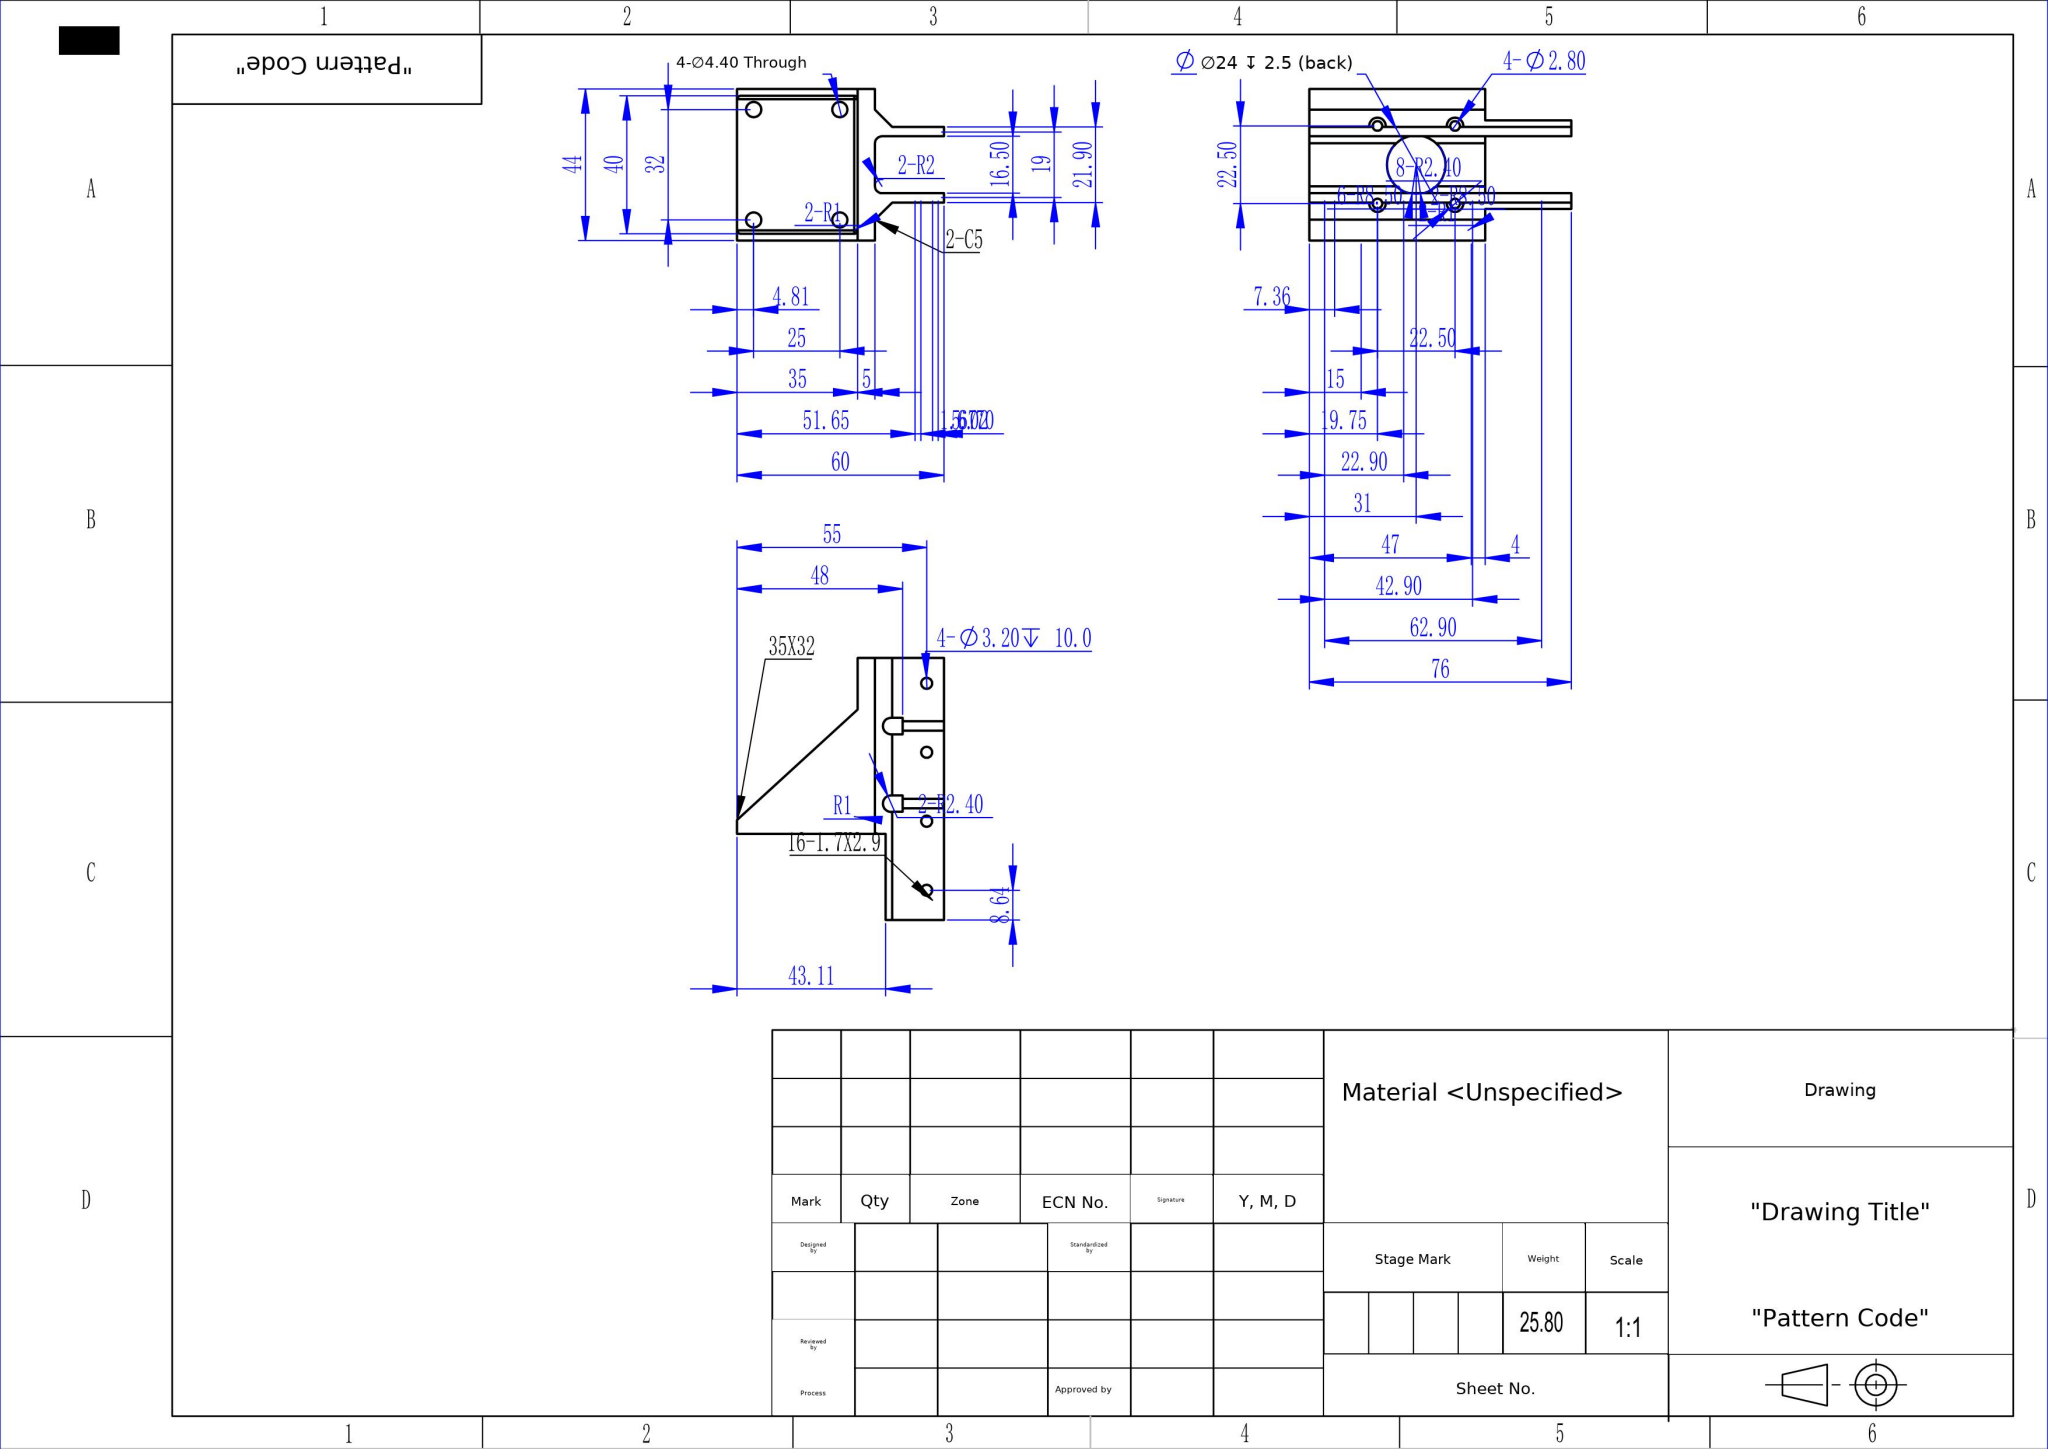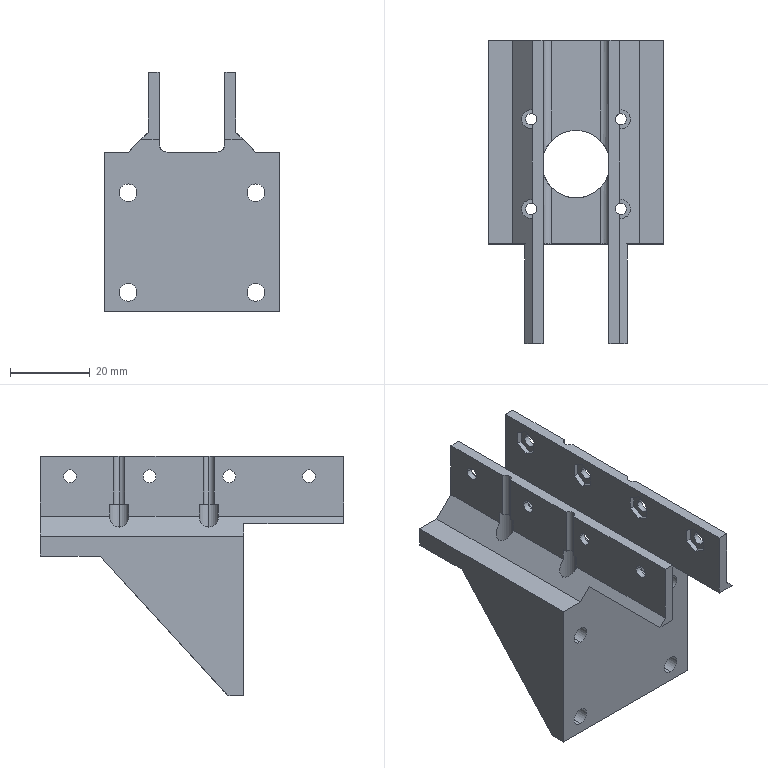Part | SolidWorks | mm | 1 solid | 159 faces | box 44 x 76 x 60 mm | volume 25803 mm3 | plane 98 | cylinder 59 | sphere 2 | commonest cylinder face diameters 3.2 x16 2.8 x14 4.4 x8 4.8 x8 2 x5 4 x4 24 x2 17 x2